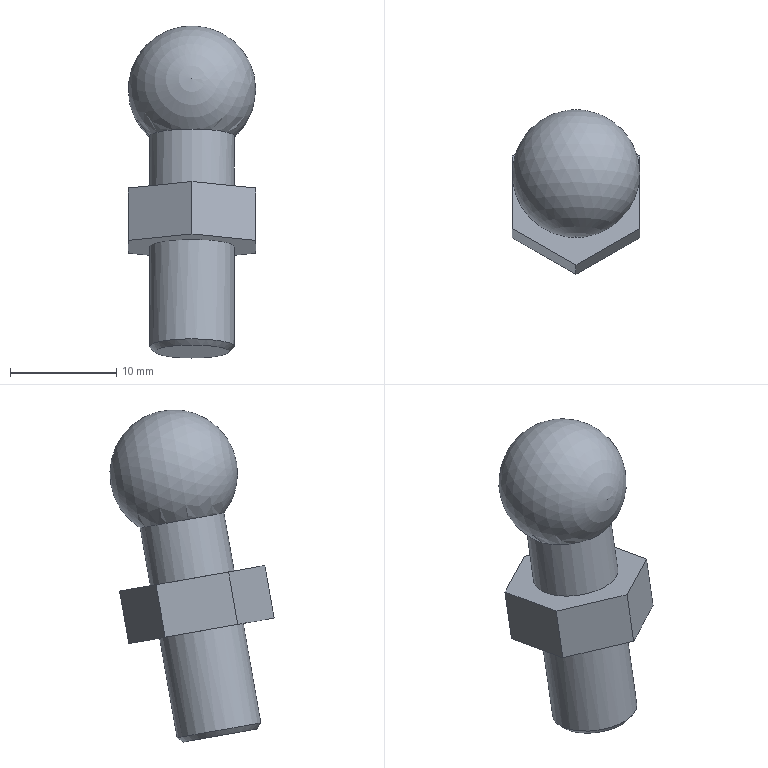Component | NX | BALL_JOINT_SCREW | 1 solid | 13 faces | box 12 x 15.43 x 31.23 mm | volume 2266 mm3 | plane 9 | cylinder 2 | sphere 1 | cone 1 | commonest cylinder face diameters 8 x2
STEP:
#1=CARTESIAN_POINT('',(0.,0.,0.));
#2=DIRECTION('',(0.,0.,1.));
#3=DIRECTION('',(1.,0.,0.));
#4=AXIS2_PLACEMENT_3D('',#1,#2,#3);
#5=CARTESIAN_POINT('',(102.166,147.569,85.412));
#6=VERTEX_POINT('',#5);
#7=CARTESIAN_POINT('',(102.166,151.508,84.718));
#8=DIRECTION('',(0.,0.1736,0.9848));
#9=DIRECTION('',(0.,-0.9848,0.1736));
#10=AXIS2_PLACEMENT_3D('',#7,#8,#9);
#11=CIRCLE('',#10,4.);
#12=CARTESIAN_POINT('',(102.166,150.548,79.274));
#13=DIRECTION('',(0.,0.1736,0.9848));
#14=DIRECTION('',(0.,-0.9848,0.1736));
#15=AXIS2_PLACEMENT_3D('',#12,#13,#14);
#16=CYLINDRICAL_SURFACE('',#15,4.);
#17=CARTESIAN_POINT('',(0.,5.528));
#18=DIRECTION('',(1.,0.));
#19=VECTOR('',#18,1.);
#20=LINE('',#17,#19);
#21=(GEOMETRIC_REPRESENTATION_CONTEXT(2)PARAMETRIC_REPRESENTATION_CONTEXT()REPRESENTATION_CONTEXT('',''));
#22=DEFINITIONAL_REPRESENTATION('',(#20),#21);
#23=PCURVE('',#16,#22);
#24=CARTESIAN_POINT('',(102.166,152.285,89.122));
#25=DIRECTION('',(0.,-0.9848,0.1736));
#26=DIRECTION('',(1.,0.,0.));
#27=AXIS2_PLACEMENT_3D('',#24,#25,#26);
#28=SPHERICAL_SURFACE('',#27,6.);
#29=CARTESIAN_POINT('',(4.712,0.7297));
#30=CARTESIAN_POINT('',(4.8,0.7303));
#31=CARTESIAN_POINT('',(4.966,0.7046));
#32=CARTESIAN_POINT('',(5.174,0.6029));
#33=CARTESIAN_POINT('',(5.316,0.4562));
#34=CARTESIAN_POINT('',(5.403,0.2829));
#35=CARTESIAN_POINT('',(5.444,0.09573));
#36=CARTESIAN_POINT('',(5.444,-0.09573));
#37=CARTESIAN_POINT('',(5.403,-0.2829));
#38=CARTESIAN_POINT('',(5.316,-0.4562));
#39=CARTESIAN_POINT('',(5.173,-0.6028));
#40=CARTESIAN_POINT('',(4.967,-0.7048));
#41=CARTESIAN_POINT('',(4.712,-0.7422));
#42=CARTESIAN_POINT('',(4.457,-0.7048));
#43=CARTESIAN_POINT('',(4.251,-0.6028));
#44=CARTESIAN_POINT('',(4.109,-0.4562));
#45=CARTESIAN_POINT('',(4.022,-0.2829));
#46=CARTESIAN_POINT('',(3.981,-0.09573));
#47=CARTESIAN_POINT('',(3.981,0.09573));
#48=CARTESIAN_POINT('',(4.022,0.2829));
#49=CARTESIAN_POINT('',(4.109,0.4562));
#50=CARTESIAN_POINT('',(4.251,0.6029));
#51=CARTESIAN_POINT('',(4.459,0.7046));
#52=CARTESIAN_POINT('',(4.625,0.7303));
#53=CARTESIAN_POINT('',(4.712,0.7297));
#54=B_SPLINE_CURVE_WITH_KNOTS('',3,(#29,#30,#31,#32,#33,#34,#35,#36,#37,#38,#39,#40,#41,#42,#43,#44,#45,#46,#47,#48,#49,#50,#51,#52,#53),.UNSPECIFIED.,.T.,.F.,(4,1,1,1,1,1,1,1,1,1,1,1,1,1,1,1,1,1,1,1,1,1,4),(0.,0.2856,0.5712,0.8568,1.142,1.428,1.714,1.999,2.285,2.57,2.856,3.142,3.427,3.713,3.998,4.284,4.57,4.855,5.141,5.426,5.712,5.998,6.283),.QUASI_UNIFORM_KNOTS.);
#55=(GEOMETRIC_REPRESENTATION_CONTEXT(2)PARAMETRIC_REPRESENTATION_CONTEXT()REPRESENTATION_CONTEXT('',''));
#56=DEFINITIONAL_REPRESENTATION('',(#54),#55);
#57=PCURVE('',#28,#56);
#58=SURFACE_CURVE('',#11,(#23,#57),.PCURVE_S1.);
#59=EDGE_CURVE('',#6,#6,#58,.T.);
#60=ORIENTED_EDGE('',*,*,#59,.F.);
#61=CARTESIAN_POINT('',(102.166,146.609,79.968));
#62=VERTEX_POINT('',#61);
#63=CARTESIAN_POINT('',(102.166,146.609,79.968));
#64=CARTESIAN_POINT('',(102.166,147.569,85.412));
#65=B_SPLINE_CURVE_WITH_KNOTS('',1,(#63,#64),.UNSPECIFIED.,.F.,.F.,(2,2),(0.,5.528),.PIECEWISE_BEZIER_KNOTS.);
#66=CARTESIAN_POINT('',(0.,0.));
#67=DIRECTION('',(0.,1.));
#68=VECTOR('',#67,1.);
#69=LINE('',#66,#68);
#70=(GEOMETRIC_REPRESENTATION_CONTEXT(2)PARAMETRIC_REPRESENTATION_CONTEXT()REPRESENTATION_CONTEXT('',''));
#71=DEFINITIONAL_REPRESENTATION('',(#69),#70);
#72=PCURVE('',#16,#71);
#73=CARTESIAN_POINT('',(6.283,0.));
#74=DIRECTION('',(0.,1.));
#75=VECTOR('',#74,1.);
#76=LINE('',#73,#75);
#77=(GEOMETRIC_REPRESENTATION_CONTEXT(2)PARAMETRIC_REPRESENTATION_CONTEXT()REPRESENTATION_CONTEXT('',''));
#78=DEFINITIONAL_REPRESENTATION('',(#76),#77);
#79=PCURVE('',#16,#78);
#80=SEAM_CURVE('',#65,(#72,#79),.PCURVE_S1.);
#81=EDGE_CURVE('',#62,#6,#80,.T.);
#82=ORIENTED_EDGE('',*,*,#81,.F.);
#83=CARTESIAN_POINT('',(106.166,150.548,79.274));
#84=VERTEX_POINT('',#83);
#85=CARTESIAN_POINT('',(102.166,150.548,79.274));
#86=DIRECTION('',(0.,-0.1736,-0.9848));
#87=DIRECTION('',(1.,0.,0.));
#88=AXIS2_PLACEMENT_3D('',#85,#86,#87);
#89=CIRCLE('',#88,4.);
#90=CARTESIAN_POINT('',(1.571,0.));
#91=DIRECTION('',(-1.,0.));
#92=VECTOR('',#91,1.);
#93=LINE('',#90,#92);
#94=(GEOMETRIC_REPRESENTATION_CONTEXT(2)PARAMETRIC_REPRESENTATION_CONTEXT()REPRESENTATION_CONTEXT('',''));
#95=DEFINITIONAL_REPRESENTATION('',(#93),#94);
#96=PCURVE('',#16,#95);
#97=CARTESIAN_POINT('',(102.166,150.548,79.274));
#98=DIRECTION('',(0.,-0.1736,-0.9848));
#99=DIRECTION('',(0.,0.9848,-0.1736));
#100=AXIS2_PLACEMENT_3D('',#97,#98,#99);
#101=PLANE('',#100);
#102=CARTESIAN_POINT('',(0.,0.));
#103=DIRECTION('',(0.,1.));
#104=AXIS2_PLACEMENT_2D('',#102,#103);
#105=CIRCLE('',#104,4.);
#106=(GEOMETRIC_REPRESENTATION_CONTEXT(2)PARAMETRIC_REPRESENTATION_CONTEXT()REPRESENTATION_CONTEXT('',''));
#107=DEFINITIONAL_REPRESENTATION('',(#105),#106);
#108=PCURVE('',#101,#107);
#109=SURFACE_CURVE('',#89,(#96,#108),.PCURVE_S1.);
#110=EDGE_CURVE('',#84,#62,#109,.T.);
#111=ORIENTED_EDGE('',*,*,#110,.F.);
#112=CARTESIAN_POINT('',(102.166,150.548,79.274));
#113=DIRECTION('',(0.,-0.1736,-0.9848));
#114=DIRECTION('',(1.,0.,0.));
#115=AXIS2_PLACEMENT_3D('',#112,#113,#114);
#116=CIRCLE('',#115,4.);
#117=CARTESIAN_POINT('',(7.854,0.));
#118=DIRECTION('',(-1.,0.));
#119=VECTOR('',#118,1.);
#120=LINE('',#117,#119);
#121=(GEOMETRIC_REPRESENTATION_CONTEXT(2)PARAMETRIC_REPRESENTATION_CONTEXT()REPRESENTATION_CONTEXT('',''));
#122=DEFINITIONAL_REPRESENTATION('',(#120),#121);
#123=PCURVE('',#16,#122);
#124=CARTESIAN_POINT('',(0.,0.));
#125=DIRECTION('',(0.,1.));
#126=AXIS2_PLACEMENT_2D('',#124,#125);
#127=CIRCLE('',#126,4.);
#128=(GEOMETRIC_REPRESENTATION_CONTEXT(2)PARAMETRIC_REPRESENTATION_CONTEXT()REPRESENTATION_CONTEXT('',''));
#129=DEFINITIONAL_REPRESENTATION('',(#127),#128);
#130=PCURVE('',#101,#129);
#131=SURFACE_CURVE('',#116,(#123,#130),.PCURVE_S1.);
#132=EDGE_CURVE('',#62,#84,#131,.T.);
#133=ORIENTED_EDGE('',*,*,#132,.F.);
#134=ORIENTED_EDGE('',*,*,#81,.T.);
#135=EDGE_LOOP('',(#60,#82,#111,#133,#134));
#136=FACE_BOUND('',#135,.T.);
#137=ADVANCED_FACE('',(#136),#16,.T.);
#138=ORIENTED_EDGE('',*,*,#59,.T.);
#139=EDGE_LOOP('',(#138));
#140=FACE_BOUND('',#139,.T.);
#141=CARTESIAN_POINT('',(102.166,158.194,88.08));
#142=VERTEX_POINT('',#141);
#143=VERTEX_LOOP('',#142);
#144=FACE_BOUND('',#143,.T.);
#145=ADVANCED_FACE('',(#140,#144),#28,.T.);
#146=CARTESIAN_POINT('',(96.166,147.137,79.875));
#147=VERTEX_POINT('',#146);
#148=CARTESIAN_POINT('',(96.166,153.96,78.672));
#149=VERTEX_POINT('',#148);
#150=CARTESIAN_POINT('',(96.166,147.137,79.875));
#151=DIRECTION('',(0.,0.9848,-0.1736));
#152=VECTOR('',#151,1.);
#153=LINE('',#150,#152);
#154=CARTESIAN_POINT('',(96.166,146.269,74.951));
#155=DIRECTION('',(1.,0.,0.));
#156=DIRECTION('',(0.,0.9848,-0.1736));
#157=AXIS2_PLACEMENT_3D('',#154,#155,#156);
#158=PLANE('',#157);
#159=CARTESIAN_POINT('',(0.,5.));
#160=DIRECTION('',(1.,0.));
#161=VECTOR('',#160,1.);
#162=LINE('',#159,#161);
#163=(GEOMETRIC_REPRESENTATION_CONTEXT(2)PARAMETRIC_REPRESENTATION_CONTEXT()REPRESENTATION_CONTEXT('',''));
#164=DEFINITIONAL_REPRESENTATION('',(#162),#163);
#165=PCURVE('',#158,#164);
#166=CARTESIAN_POINT('',(-3.464,-6.));
#167=DIRECTION('',(1.,0.));
#168=VECTOR('',#167,1.);
#169=LINE('',#166,#168);
#170=(GEOMETRIC_REPRESENTATION_CONTEXT(2)PARAMETRIC_REPRESENTATION_CONTEXT()REPRESENTATION_CONTEXT('',''));
#171=DEFINITIONAL_REPRESENTATION('',(#169),#170);
#172=PCURVE('',#101,#171);
#173=SURFACE_CURVE('',#153,(#165,#172),.PCURVE_S1.);
#174=EDGE_CURVE('',#147,#149,#173,.T.);
#175=ORIENTED_EDGE('',*,*,#174,.T.);
#176=CARTESIAN_POINT('',(96.166,153.092,73.748));
#177=VERTEX_POINT('',#176);
#178=CARTESIAN_POINT('',(96.166,153.092,73.748));
#179=DIRECTION('',(0.,0.1736,0.9848));
#180=VECTOR('',#179,1.);
#181=LINE('',#178,#180);
#182=CARTESIAN_POINT('',(6.928,0.));
#183=DIRECTION('',(0.,1.));
#184=VECTOR('',#183,1.);
#185=LINE('',#182,#184);
#186=(GEOMETRIC_REPRESENTATION_CONTEXT(2)PARAMETRIC_REPRESENTATION_CONTEXT()REPRESENTATION_CONTEXT('',''));
#187=DEFINITIONAL_REPRESENTATION('',(#185),#186);
#188=PCURVE('',#158,#187);
#189=CARTESIAN_POINT('',(96.166,153.092,73.748));
#190=DIRECTION('',(0.5,-0.8529,0.1504));
#191=DIRECTION('',(0.866,0.4924,-0.08682));
#192=AXIS2_PLACEMENT_3D('',#189,#190,#191);
#193=PLANE('',#192);
#194=CARTESIAN_POINT('',(0.,0.));
#195=DIRECTION('',(0.,1.));
#196=VECTOR('',#195,1.);
#197=LINE('',#194,#196);
#198=(GEOMETRIC_REPRESENTATION_CONTEXT(2)PARAMETRIC_REPRESENTATION_CONTEXT()REPRESENTATION_CONTEXT('',''));
#199=DEFINITIONAL_REPRESENTATION('',(#197),#198);
#200=PCURVE('',#193,#199);
#201=SURFACE_CURVE('',#181,(#188,#200),.PCURVE_S1.);
#202=EDGE_CURVE('',#177,#149,#201,.T.);
#203=ORIENTED_EDGE('',*,*,#202,.F.);
#204=CARTESIAN_POINT('',(96.166,146.269,74.951));
#205=VERTEX_POINT('',#204);
#206=CARTESIAN_POINT('',(96.166,146.269,74.951));
#207=DIRECTION('',(0.,0.9848,-0.1736));
#208=VECTOR('',#207,1.);
#209=LINE('',#206,#208);
#210=CARTESIAN_POINT('',(0.,0.));
#211=DIRECTION('',(1.,0.));
#212=VECTOR('',#211,1.);
#213=LINE('',#210,#212);
#214=(GEOMETRIC_REPRESENTATION_CONTEXT(2)PARAMETRIC_REPRESENTATION_CONTEXT()REPRESENTATION_CONTEXT('',''));
#215=DEFINITIONAL_REPRESENTATION('',(#213),#214);
#216=PCURVE('',#158,#215);
#217=CARTESIAN_POINT('',(102.166,149.68,74.35));
#218=DIRECTION('',(0.,-0.1736,-0.9848));
#219=DIRECTION('',(0.,0.9848,-0.1736));
#220=AXIS2_PLACEMENT_3D('',#217,#218,#219);
#221=PLANE('',#220);
#222=CARTESIAN_POINT('',(-3.464,-6.));
#223=DIRECTION('',(1.,0.));
#224=VECTOR('',#223,1.);
#225=LINE('',#222,#224);
#226=(GEOMETRIC_REPRESENTATION_CONTEXT(2)PARAMETRIC_REPRESENTATION_CONTEXT()REPRESENTATION_CONTEXT('',''));
#227=DEFINITIONAL_REPRESENTATION('',(#225),#226);
#228=PCURVE('',#221,#227);
#229=SURFACE_CURVE('',#209,(#216,#228),.PCURVE_S1.);
#230=EDGE_CURVE('',#205,#177,#229,.T.);
#231=ORIENTED_EDGE('',*,*,#230,.F.);
#232=CARTESIAN_POINT('',(96.166,146.269,74.951));
#233=DIRECTION('',(0.,0.1736,0.9848));
#234=VECTOR('',#233,1.);
#235=LINE('',#232,#234);
#236=CARTESIAN_POINT('',(0.,0.));
#237=DIRECTION('',(0.,1.));
#238=VECTOR('',#237,1.);
#239=LINE('',#236,#238);
#240=(GEOMETRIC_REPRESENTATION_CONTEXT(2)PARAMETRIC_REPRESENTATION_CONTEXT()REPRESENTATION_CONTEXT('',''));
#241=DEFINITIONAL_REPRESENTATION('',(#239),#240);
#242=PCURVE('',#158,#241);
#243=CARTESIAN_POINT('',(102.166,142.857,75.553));
#244=DIRECTION('',(0.5,0.8529,-0.1504));
#245=DIRECTION('',(-0.866,0.4924,-0.08682));
#246=AXIS2_PLACEMENT_3D('',#243,#244,#245);
#247=PLANE('',#246);
#248=CARTESIAN_POINT('',(6.928,-0.));
#249=DIRECTION('',(0.,1.));
#250=VECTOR('',#249,1.);
#251=LINE('',#248,#250);
#252=(GEOMETRIC_REPRESENTATION_CONTEXT(2)PARAMETRIC_REPRESENTATION_CONTEXT()REPRESENTATION_CONTEXT('',''));
#253=DEFINITIONAL_REPRESENTATION('',(#251),#252);
#254=PCURVE('',#247,#253);
#255=SURFACE_CURVE('',#235,(#242,#254),.PCURVE_S1.);
#256=EDGE_CURVE('',#205,#147,#255,.T.);
#257=ORIENTED_EDGE('',*,*,#256,.T.);
#258=EDGE_LOOP('',(#175,#203,#231,#257));
#259=FACE_BOUND('',#258,.T.);
#260=ADVANCED_FACE('',(#259),#158,.F.);
#261=CARTESIAN_POINT('',(102.166,157.371,78.071));
#262=VERTEX_POINT('',#261);
#263=CARTESIAN_POINT('',(96.166,153.96,78.672));
#264=DIRECTION('',(0.866,0.4924,-0.08682));
#265=VECTOR('',#264,1.);
#266=LINE('',#263,#265);
#267=CARTESIAN_POINT('',(0.,5.));
#268=DIRECTION('',(1.,0.));
#269=VECTOR('',#268,1.);
#270=LINE('',#267,#269);
#271=(GEOMETRIC_REPRESENTATION_CONTEXT(2)PARAMETRIC_REPRESENTATION_CONTEXT()REPRESENTATION_CONTEXT('',''));
#272=DEFINITIONAL_REPRESENTATION('',(#270),#271);
#273=PCURVE('',#193,#272);
#274=CARTESIAN_POINT('',(3.464,-6.));
#275=DIRECTION('',(0.5,0.866));
#276=VECTOR('',#275,1.);
#277=LINE('',#274,#276);
#278=(GEOMETRIC_REPRESENTATION_CONTEXT(2)PARAMETRIC_REPRESENTATION_CONTEXT()REPRESENTATION_CONTEXT('',''));
#279=DEFINITIONAL_REPRESENTATION('',(#277),#278);
#280=PCURVE('',#101,#279);
#281=SURFACE_CURVE('',#266,(#273,#280),.PCURVE_S1.);
#282=EDGE_CURVE('',#149,#262,#281,.T.);
#283=ORIENTED_EDGE('',*,*,#282,.T.);
#284=CARTESIAN_POINT('',(102.166,156.503,73.147));
#285=VERTEX_POINT('',#284);
#286=CARTESIAN_POINT('',(102.166,156.503,73.147));
#287=DIRECTION('',(0.,0.1736,0.9848));
#288=VECTOR('',#287,1.);
#289=LINE('',#286,#288);
#290=CARTESIAN_POINT('',(6.928,0.));
#291=DIRECTION('',(0.,1.));
#292=VECTOR('',#291,1.);
#293=LINE('',#290,#292);
#294=(GEOMETRIC_REPRESENTATION_CONTEXT(2)PARAMETRIC_REPRESENTATION_CONTEXT()REPRESENTATION_CONTEXT('',''));
#295=DEFINITIONAL_REPRESENTATION('',(#293),#294);
#296=PCURVE('',#193,#295);
#297=CARTESIAN_POINT('',(102.166,156.503,73.147));
#298=DIRECTION('',(-0.5,-0.8529,0.1504));
#299=DIRECTION('',(0.866,-0.4924,0.08682));
#300=AXIS2_PLACEMENT_3D('',#297,#298,#299);
#301=PLANE('',#300);
#302=CARTESIAN_POINT('',(0.,0.));
#303=DIRECTION('',(-0.,1.));
#304=VECTOR('',#303,1.);
#305=LINE('',#302,#304);
#306=(GEOMETRIC_REPRESENTATION_CONTEXT(2)PARAMETRIC_REPRESENTATION_CONTEXT()REPRESENTATION_CONTEXT('',''));
#307=DEFINITIONAL_REPRESENTATION('',(#305),#306);
#308=PCURVE('',#301,#307);
#309=SURFACE_CURVE('',#289,(#296,#308),.PCURVE_S1.);
#310=EDGE_CURVE('',#285,#262,#309,.T.);
#311=ORIENTED_EDGE('',*,*,#310,.F.);
#312=CARTESIAN_POINT('',(96.166,153.092,73.748));
#313=DIRECTION('',(0.866,0.4924,-0.08682));
#314=VECTOR('',#313,1.);
#315=LINE('',#312,#314);
#316=CARTESIAN_POINT('',(0.,0.));
#317=DIRECTION('',(1.,0.));
#318=VECTOR('',#317,1.);
#319=LINE('',#316,#318);
#320=(GEOMETRIC_REPRESENTATION_CONTEXT(2)PARAMETRIC_REPRESENTATION_CONTEXT()REPRESENTATION_CONTEXT('',''));
#321=DEFINITIONAL_REPRESENTATION('',(#319),#320);
#322=PCURVE('',#193,#321);
#323=CARTESIAN_POINT('',(3.464,-6.));
#324=DIRECTION('',(0.5,0.866));
#325=VECTOR('',#324,1.);
#326=LINE('',#323,#325);
#327=(GEOMETRIC_REPRESENTATION_CONTEXT(2)PARAMETRIC_REPRESENTATION_CONTEXT()REPRESENTATION_CONTEXT('',''));
#328=DEFINITIONAL_REPRESENTATION('',(#326),#327);
#329=PCURVE('',#221,#328);
#330=SURFACE_CURVE('',#315,(#322,#329),.PCURVE_S1.);
#331=EDGE_CURVE('',#177,#285,#330,.T.);
#332=ORIENTED_EDGE('',*,*,#331,.F.);
#333=ORIENTED_EDGE('',*,*,#202,.T.);
#334=EDGE_LOOP('',(#283,#311,#332,#333));
#335=FACE_BOUND('',#334,.T.);
#336=ADVANCED_FACE('',(#335),#193,.F.);
#337=CARTESIAN_POINT('',(108.166,153.96,78.672));
#338=VERTEX_POINT('',#337);
#339=CARTESIAN_POINT('',(102.166,157.371,78.071));
#340=DIRECTION('',(0.866,-0.4924,0.08682));
#341=VECTOR('',#340,1.);
#342=LINE('',#339,#341);
#343=CARTESIAN_POINT('',(0.,5.));
#344=DIRECTION('',(1.,-0.));
#345=VECTOR('',#344,1.);
#346=LINE('',#343,#345);
#347=(GEOMETRIC_REPRESENTATION_CONTEXT(2)PARAMETRIC_REPRESENTATION_CONTEXT()REPRESENTATION_CONTEXT('',''));
#348=DEFINITIONAL_REPRESENTATION('',(#346),#347);
#349=PCURVE('',#301,#348);
#350=CARTESIAN_POINT('',(6.928,0.));
#351=DIRECTION('',(-0.5,0.866));
#352=VECTOR('',#351,1.);
#353=LINE('',#350,#352);
#354=(GEOMETRIC_REPRESENTATION_CONTEXT(2)PARAMETRIC_REPRESENTATION_CONTEXT()REPRESENTATION_CONTEXT('',''));
#355=DEFINITIONAL_REPRESENTATION('',(#353),#354);
#356=PCURVE('',#101,#355);
#357=SURFACE_CURVE('',#342,(#349,#356),.PCURVE_S1.);
#358=EDGE_CURVE('',#262,#338,#357,.T.);
#359=ORIENTED_EDGE('',*,*,#358,.T.);
#360=CARTESIAN_POINT('',(108.166,153.092,73.748));
#361=VERTEX_POINT('',#360);
#362=CARTESIAN_POINT('',(108.166,153.092,73.748));
#363=DIRECTION('',(0.,0.1736,0.9848));
#364=VECTOR('',#363,1.);
#365=LINE('',#362,#364);
#366=CARTESIAN_POINT('',(6.928,-0.));
#367=DIRECTION('',(-0.,1.));
#368=VECTOR('',#367,1.);
#369=LINE('',#366,#368);
#370=(GEOMETRIC_REPRESENTATION_CONTEXT(2)PARAMETRIC_REPRESENTATION_CONTEXT()REPRESENTATION_CONTEXT('',''));
#371=DEFINITIONAL_REPRESENTATION('',(#369),#370);
#372=PCURVE('',#301,#371);
#373=CARTESIAN_POINT('',(108.166,153.092,73.748));
#374=DIRECTION('',(-1.,-0.,0.));
#375=DIRECTION('',(0.,-0.9848,0.1736));
#376=AXIS2_PLACEMENT_3D('',#373,#374,#375);
#377=PLANE('',#376);
#378=CARTESIAN_POINT('',(0.,0.));
#379=DIRECTION('',(0.,1.));
#380=VECTOR('',#379,1.);
#381=LINE('',#378,#380);
#382=(GEOMETRIC_REPRESENTATION_CONTEXT(2)PARAMETRIC_REPRESENTATION_CONTEXT()REPRESENTATION_CONTEXT('',''));
#383=DEFINITIONAL_REPRESENTATION('',(#381),#382);
#384=PCURVE('',#377,#383);
#385=SURFACE_CURVE('',#365,(#372,#384),.PCURVE_S1.);
#386=EDGE_CURVE('',#361,#338,#385,.T.);
#387=ORIENTED_EDGE('',*,*,#386,.F.);
#388=CARTESIAN_POINT('',(102.166,156.503,73.147));
#389=DIRECTION('',(0.866,-0.4924,0.08682));
#390=VECTOR('',#389,1.);
#391=LINE('',#388,#390);
#392=CARTESIAN_POINT('',(0.,0.));
#393=DIRECTION('',(1.,-0.));
#394=VECTOR('',#393,1.);
#395=LINE('',#392,#394);
#396=(GEOMETRIC_REPRESENTATION_CONTEXT(2)PARAMETRIC_REPRESENTATION_CONTEXT()REPRESENTATION_CONTEXT('',''));
#397=DEFINITIONAL_REPRESENTATION('',(#395),#396);
#398=PCURVE('',#301,#397);
#399=CARTESIAN_POINT('',(6.928,0.));
#400=DIRECTION('',(-0.5,0.866));
#401=VECTOR('',#400,1.);
#402=LINE('',#399,#401);
#403=(GEOMETRIC_REPRESENTATION_CONTEXT(2)PARAMETRIC_REPRESENTATION_CONTEXT()REPRESENTATION_CONTEXT('',''));
#404=DEFINITIONAL_REPRESENTATION('',(#402),#403);
#405=PCURVE('',#221,#404);
#406=SURFACE_CURVE('',#391,(#398,#405),.PCURVE_S1.);
#407=EDGE_CURVE('',#285,#361,#406,.T.);
#408=ORIENTED_EDGE('',*,*,#407,.F.);
#409=ORIENTED_EDGE('',*,*,#310,.T.);
#410=EDGE_LOOP('',(#359,#387,#408,#409));
#411=FACE_BOUND('',#410,.T.);
#412=ADVANCED_FACE('',(#411),#301,.F.);
#413=CARTESIAN_POINT('',(108.166,147.137,79.875));
#414=VERTEX_POINT('',#413);
#415=CARTESIAN_POINT('',(108.166,153.96,78.672));
#416=DIRECTION('',(0.,-0.9848,0.1736));
#417=VECTOR('',#416,1.);
#418=LINE('',#415,#417);
#419=CARTESIAN_POINT('',(-0.,5.));
#420=DIRECTION('',(1.,0.));
#421=VECTOR('',#420,1.);
#422=LINE('',#419,#421);
#423=(GEOMETRIC_REPRESENTATION_CONTEXT(2)PARAMETRIC_REPRESENTATION_CONTEXT()REPRESENTATION_CONTEXT('',''));
#424=DEFINITIONAL_REPRESENTATION('',(#422),#423);
#425=PCURVE('',#377,#424);
#426=CARTESIAN_POINT('',(3.464,6.));
#427=DIRECTION('',(-1.,0.));
#428=VECTOR('',#427,1.);
#429=LINE('',#426,#428);
#430=(GEOMETRIC_REPRESENTATION_CONTEXT(2)PARAMETRIC_REPRESENTATION_CONTEXT()REPRESENTATION_CONTEXT('',''));
#431=DEFINITIONAL_REPRESENTATION('',(#429),#430);
#432=PCURVE('',#101,#431);
#433=SURFACE_CURVE('',#418,(#425,#432),.PCURVE_S1.);
#434=EDGE_CURVE('',#338,#414,#433,.T.);
#435=ORIENTED_EDGE('',*,*,#434,.T.);
#436=CARTESIAN_POINT('',(108.166,146.269,74.951));
#437=VERTEX_POINT('',#436);
#438=CARTESIAN_POINT('',(108.166,146.269,74.951));
#439=DIRECTION('',(0.,0.1736,0.9848));
#440=VECTOR('',#439,1.);
#441=LINE('',#438,#440);
#442=CARTESIAN_POINT('',(6.928,-0.));
#443=DIRECTION('',(0.,1.));
#444=VECTOR('',#443,1.);
#445=LINE('',#442,#444);
#446=(GEOMETRIC_REPRESENTATION_CONTEXT(2)PARAMETRIC_REPRESENTATION_CONTEXT()REPRESENTATION_CONTEXT('',''));
#447=DEFINITIONAL_REPRESENTATION('',(#445),#446);
#448=PCURVE('',#377,#447);
#449=CARTESIAN_POINT('',(108.166,146.269,74.951));
#450=DIRECTION('',(-0.5,0.8529,-0.1504));
#451=DIRECTION('',(-0.866,-0.4924,0.08682));
#452=AXIS2_PLACEMENT_3D('',#449,#450,#451);
#453=PLANE('',#452);
#454=CARTESIAN_POINT('',(0.,0.));
#455=DIRECTION('',(-0.,1.));
#456=VECTOR('',#455,1.);
#457=LINE('',#454,#456);
#458=(GEOMETRIC_REPRESENTATION_CONTEXT(2)PARAMETRIC_REPRESENTATION_CONTEXT()REPRESENTATION_CONTEXT('',''));
#459=DEFINITIONAL_REPRESENTATION('',(#457),#458);
#460=PCURVE('',#453,#459);
#461=SURFACE_CURVE('',#441,(#448,#460),.PCURVE_S1.);
#462=EDGE_CURVE('',#437,#414,#461,.T.);
#463=ORIENTED_EDGE('',*,*,#462,.F.);
#464=CARTESIAN_POINT('',(108.166,153.092,73.748));
#465=DIRECTION('',(0.,-0.9848,0.1736));
#466=VECTOR('',#465,1.);
#467=LINE('',#464,#466);
#468=CARTESIAN_POINT('',(0.,0.));
#469=DIRECTION('',(1.,0.));
#470=VECTOR('',#469,1.);
#471=LINE('',#468,#470);
#472=(GEOMETRIC_REPRESENTATION_CONTEXT(2)PARAMETRIC_REPRESENTATION_CONTEXT()REPRESENTATION_CONTEXT('',''));
#473=DEFINITIONAL_REPRESENTATION('',(#471),#472);
#474=PCURVE('',#377,#473);
#475=CARTESIAN_POINT('',(3.464,6.));
#476=DIRECTION('',(-1.,0.));
#477=VECTOR('',#476,1.);
#478=LINE('',#475,#477);
#479=(GEOMETRIC_REPRESENTATION_CONTEXT(2)PARAMETRIC_REPRESENTATION_CONTEXT()REPRESENTATION_CONTEXT('',''));
#480=DEFINITIONAL_REPRESENTATION('',(#478),#479);
#481=PCURVE('',#221,#480);
#482=SURFACE_CURVE('',#467,(#474,#481),.PCURVE_S1.);
#483=EDGE_CURVE('',#361,#437,#482,.T.);
#484=ORIENTED_EDGE('',*,*,#483,.F.);
#485=ORIENTED_EDGE('',*,*,#386,.T.);
#486=EDGE_LOOP('',(#435,#463,#484,#485));
#487=FACE_BOUND('',#486,.T.);
#488=ADVANCED_FACE('',(#487),#377,.F.);
#489=CARTESIAN_POINT('',(102.166,143.725,80.477));
#490=VERTEX_POINT('',#489);
#491=CARTESIAN_POINT('',(108.166,147.137,79.875));
#492=DIRECTION('',(-0.866,-0.4924,0.08682));
#493=VECTOR('',#492,1.);
#494=LINE('',#491,#493);
#495=CARTESIAN_POINT('',(-0.,5.));
#496=DIRECTION('',(1.,-0.));
#497=VECTOR('',#496,1.);
#498=LINE('',#495,#497);
#499=(GEOMETRIC_REPRESENTATION_CONTEXT(2)PARAMETRIC_REPRESENTATION_CONTEXT()REPRESENTATION_CONTEXT('',''));
#500=DEFINITIONAL_REPRESENTATION('',(#498),#499);
#501=PCURVE('',#453,#500);
#502=CARTESIAN_POINT('',(-3.464,6.));
#503=DIRECTION('',(-0.5,-0.866));
#504=VECTOR('',#503,1.);
#505=LINE('',#502,#504);
#506=(GEOMETRIC_REPRESENTATION_CONTEXT(2)PARAMETRIC_REPRESENTATION_CONTEXT()REPRESENTATION_CONTEXT('',''));
#507=DEFINITIONAL_REPRESENTATION('',(#505),#506);
#508=PCURVE('',#101,#507);
#509=SURFACE_CURVE('',#494,(#501,#508),.PCURVE_S1.);
#510=EDGE_CURVE('',#414,#490,#509,.T.);
#511=ORIENTED_EDGE('',*,*,#510,.T.);
#512=CARTESIAN_POINT('',(102.166,142.857,75.553));
#513=VERTEX_POINT('',#512);
#514=CARTESIAN_POINT('',(102.166,142.857,75.553));
#515=DIRECTION('',(0.,0.1736,0.9848));
#516=VECTOR('',#515,1.);
#517=LINE('',#514,#516);
#518=CARTESIAN_POINT('',(6.928,0.));
#519=DIRECTION('',(-0.,1.));
#520=VECTOR('',#519,1.);
#521=LINE('',#518,#520);
#522=(GEOMETRIC_REPRESENTATION_CONTEXT(2)PARAMETRIC_REPRESENTATION_CONTEXT()REPRESENTATION_CONTEXT('',''));
#523=DEFINITIONAL_REPRESENTATION('',(#521),#522);
#524=PCURVE('',#453,#523);
#525=CARTESIAN_POINT('',(0.,0.));
#526=DIRECTION('',(0.,1.));
#527=VECTOR('',#526,1.);
#528=LINE('',#525,#527);
#529=(GEOMETRIC_REPRESENTATION_CONTEXT(2)PARAMETRIC_REPRESENTATION_CONTEXT()REPRESENTATION_CONTEXT('',''));
#530=DEFINITIONAL_REPRESENTATION('',(#528),#529);
#531=PCURVE('',#247,#530);
#532=SURFACE_CURVE('',#517,(#524,#531),.PCURVE_S1.);
#533=EDGE_CURVE('',#513,#490,#532,.T.);
#534=ORIENTED_EDGE('',*,*,#533,.F.);
#535=CARTESIAN_POINT('',(108.166,146.269,74.951));
#536=DIRECTION('',(-0.866,-0.4924,0.08682));
#537=VECTOR('',#536,1.);
#538=LINE('',#535,#537);
#539=CARTESIAN_POINT('',(0.,0.));
#540=DIRECTION('',(1.,-0.));
#541=VECTOR('',#540,1.);
#542=LINE('',#539,#541);
#543=(GEOMETRIC_REPRESENTATION_CONTEXT(2)PARAMETRIC_REPRESENTATION_CONTEXT()REPRESENTATION_CONTEXT('',''));
#544=DEFINITIONAL_REPRESENTATION('',(#542),#543);
#545=PCURVE('',#453,#544);
#546=CARTESIAN_POINT('',(-3.464,6.));
#547=DIRECTION('',(-0.5,-0.866));
#548=VECTOR('',#547,1.);
#549=LINE('',#546,#548);
#550=(GEOMETRIC_REPRESENTATION_CONTEXT(2)PARAMETRIC_REPRESENTATION_CONTEXT()REPRESENTATION_CONTEXT('',''));
#551=DEFINITIONAL_REPRESENTATION('',(#549),#550);
#552=PCURVE('',#221,#551);
#553=SURFACE_CURVE('',#538,(#545,#552),.PCURVE_S1.);
#554=EDGE_CURVE('',#437,#513,#553,.T.);
#555=ORIENTED_EDGE('',*,*,#554,.F.);
#556=ORIENTED_EDGE('',*,*,#462,.T.);
#557=EDGE_LOOP('',(#511,#534,#555,#556));
#558=FACE_BOUND('',#557,.T.);
#559=ADVANCED_FACE('',(#558),#453,.F.);
#560=CARTESIAN_POINT('',(102.166,143.725,80.477));
#561=DIRECTION('',(-0.866,0.4924,-0.08682));
#562=VECTOR('',#561,1.);
#563=LINE('',#560,#562);
#564=CARTESIAN_POINT('',(-0.,5.));
#565=DIRECTION('',(1.,0.));
#566=VECTOR('',#565,1.);
#567=LINE('',#564,#566);
#568=(GEOMETRIC_REPRESENTATION_CONTEXT(2)PARAMETRIC_REPRESENTATION_CONTEXT()REPRESENTATION_CONTEXT('',''));
#569=DEFINITIONAL_REPRESENTATION('',(#567),#568);
#570=PCURVE('',#247,#569);
#571=CARTESIAN_POINT('',(-6.928,0.));
#572=DIRECTION('',(0.5,-0.866));
#573=VECTOR('',#572,1.);
#574=LINE('',#571,#573);
#575=(GEOMETRIC_REPRESENTATION_CONTEXT(2)PARAMETRIC_REPRESENTATION_CONTEXT()REPRESENTATION_CONTEXT('',''));
#576=DEFINITIONAL_REPRESENTATION('',(#574),#575);
#577=PCURVE('',#101,#576);
#578=SURFACE_CURVE('',#563,(#570,#577),.PCURVE_S1.);
#579=EDGE_CURVE('',#490,#147,#578,.T.);
#580=ORIENTED_EDGE('',*,*,#579,.T.);
#581=ORIENTED_EDGE('',*,*,#256,.F.);
#582=CARTESIAN_POINT('',(102.166,142.857,75.553));
#583=DIRECTION('',(-0.866,0.4924,-0.08682));
#584=VECTOR('',#583,1.);
#585=LINE('',#582,#584);
#586=CARTESIAN_POINT('',(0.,0.));
#587=DIRECTION('',(1.,0.));
#588=VECTOR('',#587,1.);
#589=LINE('',#586,#588);
#590=(GEOMETRIC_REPRESENTATION_CONTEXT(2)PARAMETRIC_REPRESENTATION_CONTEXT()REPRESENTATION_CONTEXT('',''));
#591=DEFINITIONAL_REPRESENTATION('',(#589),#590);
#592=PCURVE('',#247,#591);
#593=CARTESIAN_POINT('',(-6.928,0.));
#594=DIRECTION('',(0.5,-0.866));
#595=VECTOR('',#594,1.);
#596=LINE('',#593,#595);
#597=(GEOMETRIC_REPRESENTATION_CONTEXT(2)PARAMETRIC_REPRESENTATION_CONTEXT()REPRESENTATION_CONTEXT('',''));
#598=DEFINITIONAL_REPRESENTATION('',(#596),#597);
#599=PCURVE('',#221,#598);
#600=SURFACE_CURVE('',#585,(#592,#599),.PCURVE_S1.);
#601=EDGE_CURVE('',#513,#205,#600,.T.);
#602=ORIENTED_EDGE('',*,*,#601,.F.);
#603=ORIENTED_EDGE('',*,*,#533,.T.);
#604=EDGE_LOOP('',(#580,#581,#602,#603));
#605=FACE_BOUND('',#604,.T.);
#606=ADVANCED_FACE('',(#605),#247,.F.);
#607=CARTESIAN_POINT('',(105.63,151.65,74.003));
#608=VERTEX_POINT('',#607);
#609=CARTESIAN_POINT('',(102.166,149.68,74.35));
#610=DIRECTION('',(0.,-0.1736,-0.9848));
#611=DIRECTION('',(0.866,0.4924,-0.08682));
#612=AXIS2_PLACEMENT_3D('',#609,#610,#611);
#613=CIRCLE('',#612,4.);
#614=CARTESIAN_POINT('',(0.,0.));
#615=DIRECTION('',(0.5,0.866));
#616=AXIS2_PLACEMENT_2D('',#614,#615);
#617=CIRCLE('',#616,4.);
#618=(GEOMETRIC_REPRESENTATION_CONTEXT(2)PARAMETRIC_REPRESENTATION_CONTEXT()REPRESENTATION_CONTEXT('',''));
#619=DEFINITIONAL_REPRESENTATION('',(#617),#618);
#620=PCURVE('',#221,#619);
#621=CARTESIAN_POINT('',(102.166,147.944,64.502));
#622=DIRECTION('',(0.,0.1736,0.9848));
#623=DIRECTION('',(0.,-0.9848,0.1736));
#624=AXIS2_PLACEMENT_3D('',#621,#622,#623);
#625=CYLINDRICAL_SURFACE('',#624,4.);
#626=CARTESIAN_POINT('',(8.378,10.));
#627=DIRECTION('',(-1.,0.));
#628=VECTOR('',#627,1.);
#629=LINE('',#626,#628);
#630=(GEOMETRIC_REPRESENTATION_CONTEXT(2)PARAMETRIC_REPRESENTATION_CONTEXT()REPRESENTATION_CONTEXT('',''));
#631=DEFINITIONAL_REPRESENTATION('',(#629),#630);
#632=PCURVE('',#625,#631);
#633=SURFACE_CURVE('',#613,(#620,#632),.PCURVE_S1.);
#634=EDGE_CURVE('',#608,#608,#633,.T.);
#635=ORIENTED_EDGE('',*,*,#634,.F.);
#636=EDGE_LOOP('',(#635));
#637=FACE_BOUND('',#636,.T.);
#638=ORIENTED_EDGE('',*,*,#230,.T.);
#639=ORIENTED_EDGE('',*,*,#331,.T.);
#640=ORIENTED_EDGE('',*,*,#407,.T.);
#641=ORIENTED_EDGE('',*,*,#483,.T.);
#642=ORIENTED_EDGE('',*,*,#554,.T.);
#643=ORIENTED_EDGE('',*,*,#601,.T.);
#644=EDGE_LOOP('',(#638,#639,#640,#641,#642,#643));
#645=FACE_BOUND('',#644,.T.);
#646=ADVANCED_FACE('',(#637,#645),#221,.T.);
#647=ORIENTED_EDGE('',*,*,#110,.T.);
#648=ORIENTED_EDGE('',*,*,#132,.T.);
#649=EDGE_LOOP('',(#647,#648));
#650=FACE_BOUND('',#649,.T.);
#651=ORIENTED_EDGE('',*,*,#174,.F.);
#652=ORIENTED_EDGE('',*,*,#579,.F.);
#653=ORIENTED_EDGE('',*,*,#510,.F.);
#654=ORIENTED_EDGE('',*,*,#434,.F.);
#655=ORIENTED_EDGE('',*,*,#358,.F.);
#656=ORIENTED_EDGE('',*,*,#282,.F.);
#657=EDGE_LOOP('',(#651,#652,#653,#654,#655,#656));
#658=FACE_BOUND('',#657,.T.);
#659=ADVANCED_FACE('',(#650,#658),#101,.F.);
#660=CARTESIAN_POINT('',(102.166,151.97,64.3));
#661=VERTEX_POINT('',#660);
#662=CARTESIAN_POINT('',(105.63,150.,64.647));
#663=VERTEX_POINT('',#662);
#664=CARTESIAN_POINT('',(102.166,148.03,64.994));
#665=DIRECTION('',(0.,0.1736,0.9848));
#666=DIRECTION('',(0.,0.9848,-0.1736));
#667=AXIS2_PLACEMENT_3D('',#664,#665,#666);
#668=CIRCLE('',#667,4.);
#669=CARTESIAN_POINT('',(3.142,0.5));
#670=DIRECTION('',(1.,0.));
#671=VECTOR('',#670,1.);
#672=LINE('',#669,#671);
#673=(GEOMETRIC_REPRESENTATION_CONTEXT(2)PARAMETRIC_REPRESENTATION_CONTEXT()REPRESENTATION_CONTEXT('',''));
#674=DEFINITIONAL_REPRESENTATION('',(#672),#673);
#675=PCURVE('',#625,#674);
#676=CARTESIAN_POINT('',(102.166,147.944,64.502));
#677=DIRECTION('',(0.,0.1736,0.9848));
#678=DIRECTION('',(0.,-0.9848,0.1736));
#679=AXIS2_PLACEMENT_3D('',#676,#677,#678);
#680=CONICAL_SURFACE('',#679,3.5,0.7854);
#681=CARTESIAN_POINT('',(3.142,0.5));
#682=DIRECTION('',(1.,0.));
#683=VECTOR('',#682,1.);
#684=LINE('',#681,#683);
#685=(GEOMETRIC_REPRESENTATION_CONTEXT(2)PARAMETRIC_REPRESENTATION_CONTEXT()REPRESENTATION_CONTEXT('',''));
#686=DEFINITIONAL_REPRESENTATION('',(#684),#685);
#687=PCURVE('',#680,#686);
#688=SURFACE_CURVE('',#668,(#675,#687),.PCURVE_S1.);
#689=EDGE_CURVE('',#661,#663,#688,.T.);
#690=ORIENTED_EDGE('',*,*,#689,.T.);
#691=CARTESIAN_POINT('',(105.63,150.,64.647));
#692=CARTESIAN_POINT('',(105.63,151.65,74.003));
#693=B_SPLINE_CURVE_WITH_KNOTS('',1,(#691,#692),.UNSPECIFIED.,.F.,.F.,(2,2),(0.5,10.),.PIECEWISE_BEZIER_KNOTS.);
#694=CARTESIAN_POINT('',(8.378,0.));
#695=DIRECTION('',(0.,1.));
#696=VECTOR('',#695,1.);
#697=LINE('',#694,#696);
#698=(GEOMETRIC_REPRESENTATION_CONTEXT(2)PARAMETRIC_REPRESENTATION_CONTEXT()REPRESENTATION_CONTEXT('',''));
#699=DEFINITIONAL_REPRESENTATION('',(#697),#698);
#700=PCURVE('',#625,#699);
#701=CARTESIAN_POINT('',(2.094,0.));
#702=DIRECTION('',(0.,1.));
#703=VECTOR('',#702,1.);
#704=LINE('',#701,#703);
#705=(GEOMETRIC_REPRESENTATION_CONTEXT(2)PARAMETRIC_REPRESENTATION_CONTEXT()REPRESENTATION_CONTEXT('',''));
#706=DEFINITIONAL_REPRESENTATION('',(#704),#705);
#707=PCURVE('',#625,#706);
#708=SEAM_CURVE('',#693,(#700,#707),.PCURVE_S1.);
#709=EDGE_CURVE('',#663,#608,#708,.T.);
#710=ORIENTED_EDGE('',*,*,#709,.T.);
#711=ORIENTED_EDGE('',*,*,#634,.T.);
#712=ORIENTED_EDGE('',*,*,#709,.F.);
#713=CARTESIAN_POINT('',(102.166,148.03,64.994));
#714=DIRECTION('',(0.,0.1736,0.9848));
#715=DIRECTION('',(0.,0.9848,-0.1736));
#716=AXIS2_PLACEMENT_3D('',#713,#714,#715);
#717=CIRCLE('',#716,4.);
#718=CARTESIAN_POINT('',(-3.142,0.5));
#719=DIRECTION('',(1.,0.));
#720=VECTOR('',#719,1.);
#721=LINE('',#718,#720);
#722=(GEOMETRIC_REPRESENTATION_CONTEXT(2)PARAMETRIC_REPRESENTATION_CONTEXT()REPRESENTATION_CONTEXT('',''));
#723=DEFINITIONAL_REPRESENTATION('',(#721),#722);
#724=PCURVE('',#625,#723);
#725=CARTESIAN_POINT('',(3.142,0.5));
#726=DIRECTION('',(1.,-0.));
#727=VECTOR('',#726,1.);
#728=LINE('',#725,#727);
#729=(GEOMETRIC_REPRESENTATION_CONTEXT(2)PARAMETRIC_REPRESENTATION_CONTEXT()REPRESENTATION_CONTEXT('',''));
#730=DEFINITIONAL_REPRESENTATION('',(#728),#729);
#731=PCURVE('',#680,#730);
#732=SURFACE_CURVE('',#717,(#724,#731),.PCURVE_S1.);
#733=EDGE_CURVE('',#663,#661,#732,.T.);
#734=ORIENTED_EDGE('',*,*,#733,.T.);
#735=EDGE_LOOP('',(#690,#710,#711,#712,#734));
#736=FACE_BOUND('',#735,.T.);
#737=ADVANCED_FACE('',(#736),#625,.T.);
#738=CARTESIAN_POINT('',(102.166,151.39,63.894));
#739=VERTEX_POINT('',#738);
#740=CARTESIAN_POINT('',(102.166,147.944,64.502));
#741=DIRECTION('',(0.,-0.1736,-0.9848));
#742=DIRECTION('',(0.,0.9848,-0.1736));
#743=AXIS2_PLACEMENT_3D('',#740,#741,#742);
#744=CIRCLE('',#743,3.5);
#745=CARTESIAN_POINT('',(102.166,147.944,64.502));
#746=DIRECTION('',(0.,-0.1736,-0.9848));
#747=DIRECTION('',(0.,0.9848,-0.1736));
#748=AXIS2_PLACEMENT_3D('',#745,#746,#747);
#749=PLANE('',#748);
#750=CARTESIAN_POINT('',(0.,0.));
#751=DIRECTION('',(1.,0.));
#752=AXIS2_PLACEMENT_2D('',#750,#751);
#753=CIRCLE('',#752,3.5);
#754=(GEOMETRIC_REPRESENTATION_CONTEXT(2)PARAMETRIC_REPRESENTATION_CONTEXT()REPRESENTATION_CONTEXT('',''));
#755=DEFINITIONAL_REPRESENTATION('',(#753),#754);
#756=PCURVE('',#749,#755);
#757=CARTESIAN_POINT('',(9.425,0.));
#758=DIRECTION('',(-1.,0.));
#759=VECTOR('',#758,1.);
#760=LINE('',#757,#759);
#761=(GEOMETRIC_REPRESENTATION_CONTEXT(2)PARAMETRIC_REPRESENTATION_CONTEXT()REPRESENTATION_CONTEXT('',''));
#762=DEFINITIONAL_REPRESENTATION('',(#760),#761);
#763=PCURVE('',#680,#762);
#764=SURFACE_CURVE('',#744,(#756,#763),.PCURVE_S1.);
#765=EDGE_CURVE('',#739,#739,#764,.T.);
#766=ORIENTED_EDGE('',*,*,#765,.T.);
#767=EDGE_LOOP('',(#766));
#768=FACE_BOUND('',#767,.T.);
#769=ADVANCED_FACE('',(#768),#749,.T.);
#770=ORIENTED_EDGE('',*,*,#689,.F.);
#771=CARTESIAN_POINT('',(102.166,151.39,63.894));
#772=CARTESIAN_POINT('',(102.166,151.97,64.3));
#773=B_SPLINE_CURVE_WITH_KNOTS('',1,(#771,#772),.UNSPECIFIED.,.F.,.F.,(2,2),(0.,0.7071),.PIECEWISE_BEZIER_KNOTS.);
#774=CARTESIAN_POINT('',(3.142,0.));
#775=DIRECTION('',(0.,1.));
#776=VECTOR('',#775,1.);
#777=LINE('',#774,#776);
#778=(GEOMETRIC_REPRESENTATION_CONTEXT(2)PARAMETRIC_REPRESENTATION_CONTEXT()REPRESENTATION_CONTEXT('',''));
#779=DEFINITIONAL_REPRESENTATION('',(#777),#778);
#780=PCURVE('',#680,#779);
#781=CARTESIAN_POINT('',(9.425,0.));
#782=DIRECTION('',(0.,1.));
#783=VECTOR('',#782,1.);
#784=LINE('',#781,#783);
#785=(GEOMETRIC_REPRESENTATION_CONTEXT(2)PARAMETRIC_REPRESENTATION_CONTEXT()REPRESENTATION_CONTEXT('',''));
#786=DEFINITIONAL_REPRESENTATION('',(#784),#785);
#787=PCURVE('',#680,#786);
#788=SEAM_CURVE('',#773,(#780,#787),.PCURVE_S1.);
#789=EDGE_CURVE('',#739,#661,#788,.T.);
#790=ORIENTED_EDGE('',*,*,#789,.F.);
#791=ORIENTED_EDGE('',*,*,#765,.F.);
#792=ORIENTED_EDGE('',*,*,#789,.T.);
#793=ORIENTED_EDGE('',*,*,#733,.F.);
#794=EDGE_LOOP('',(#770,#790,#791,#792,#793));
#795=FACE_BOUND('',#794,.T.);
#796=ADVANCED_FACE('',(#795),#680,.T.);
#797=CLOSED_SHELL('',(#137,#145,#260,#336,#412,#488,#559,#606,#646,#659,#737,#769,#796));
#798=MANIFOLD_SOLID_BREP('',#797);
#799=(LENGTH_UNIT()NAMED_UNIT(*)SI_UNIT(.MILLI.,.METRE.));
#800=UNCERTAINTY_MEASURE_WITH_UNIT(LENGTH_MEASURE(0.000002),#799,'','');
#801=(NAMED_UNIT(*)PLANE_ANGLE_UNIT()SI_UNIT($,.RADIAN.));
#802=(NAMED_UNIT(*)SI_UNIT($,.STERADIAN.)SOLID_ANGLE_UNIT());
#803=(GEOMETRIC_REPRESENTATION_CONTEXT(3)GLOBAL_UNCERTAINTY_ASSIGNED_CONTEXT((#800))GLOBAL_UNIT_ASSIGNED_CONTEXT((#799,#801,#802))REPRESENTATION_CONTEXT('',''));
#804=ADVANCED_BREP_SHAPE_REPRESENTATION('',(#4,#798),#803);